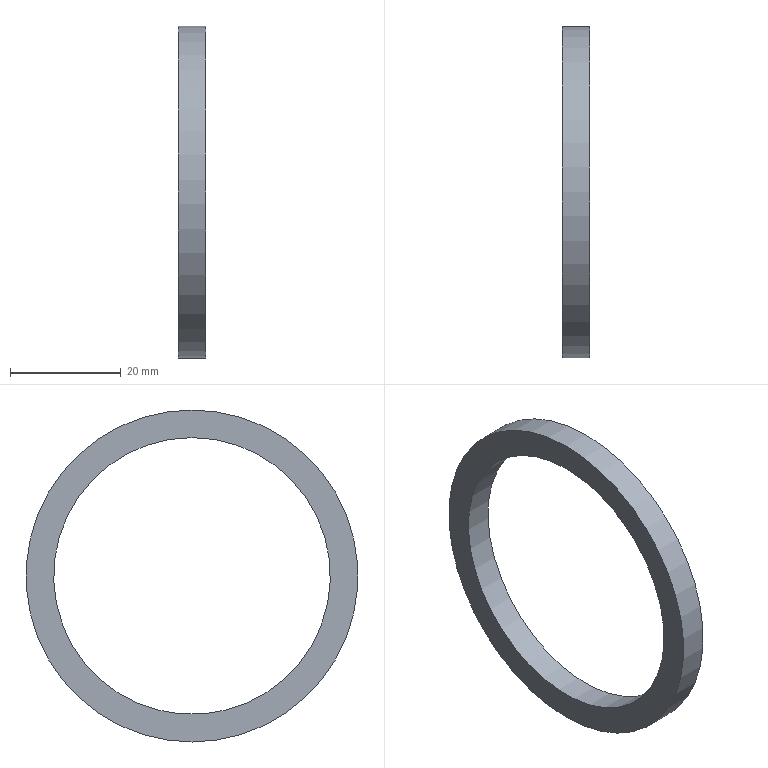Component | NX | PIN_SHAFT_WASHER | 1 solid | 4 faces | box 5 x 60 x 60 mm | volume 4320 mm3 | cylinder 2 | plane 2 | commonest cylinder face diameters 60 x1 50 x1
STEP:
#1=CARTESIAN_POINT('',(0.,0.,0.));
#2=DIRECTION('',(0.,0.,1.));
#3=DIRECTION('',(1.,0.,0.));
#4=AXIS2_PLACEMENT_3D('',#1,#2,#3);
#5=CARTESIAN_POINT('',(74.458,-1168.882,694.997));
#6=VERTEX_POINT('',#5);
#7=CARTESIAN_POINT('',(74.458,-1168.882,664.997));
#8=DIRECTION('',(1.,0.,0.));
#9=DIRECTION('',(0.,0.,1.));
#10=AXIS2_PLACEMENT_3D('',#7,#8,#9);
#11=CIRCLE('',#10,30.);
#12=CARTESIAN_POINT('',(74.458,-1168.882,664.997));
#13=DIRECTION('',(1.,0.,0.));
#14=DIRECTION('',(0.,0.,-1.));
#15=AXIS2_PLACEMENT_3D('',#12,#13,#14);
#16=CYLINDRICAL_SURFACE('',#15,30.);
#17=CARTESIAN_POINT('',(3.142,0.));
#18=DIRECTION('',(1.,0.));
#19=VECTOR('',#18,1.);
#20=LINE('',#17,#19);
#21=(GEOMETRIC_REPRESENTATION_CONTEXT(2)PARAMETRIC_REPRESENTATION_CONTEXT()REPRESENTATION_CONTEXT('',''));
#22=DEFINITIONAL_REPRESENTATION('',(#20),#21);
#23=PCURVE('',#16,#22);
#24=CARTESIAN_POINT('',(74.458,-1168.882,664.997));
#25=DIRECTION('',(1.,0.,0.));
#26=DIRECTION('',(0.,0.,-1.));
#27=AXIS2_PLACEMENT_3D('',#24,#25,#26);
#28=PLANE('',#27);
#29=CARTESIAN_POINT('',(0.,0.));
#30=DIRECTION('',(-1.,0.));
#31=AXIS2_PLACEMENT_2D('',#29,#30);
#32=CIRCLE('',#31,30.);
#33=(GEOMETRIC_REPRESENTATION_CONTEXT(2)PARAMETRIC_REPRESENTATION_CONTEXT()REPRESENTATION_CONTEXT('',''));
#34=DEFINITIONAL_REPRESENTATION('',(#32),#33);
#35=PCURVE('',#28,#34);
#36=SURFACE_CURVE('',#11,(#23,#35),.PCURVE_S1.);
#37=EDGE_CURVE('',#6,#6,#36,.T.);
#38=ORIENTED_EDGE('',*,*,#37,.T.);
#39=CARTESIAN_POINT('',(79.458,-1168.882,694.997));
#40=VERTEX_POINT('',#39);
#41=CARTESIAN_POINT('',(74.458,-1168.882,694.997));
#42=CARTESIAN_POINT('',(79.458,-1168.882,694.997));
#43=B_SPLINE_CURVE_WITH_KNOTS('',1,(#41,#42),.UNSPECIFIED.,.F.,.F.,(2,2),(0.,5.),.PIECEWISE_BEZIER_KNOTS.);
#44=CARTESIAN_POINT('',(9.425,0.));
#45=DIRECTION('',(0.,1.));
#46=VECTOR('',#45,1.);
#47=LINE('',#44,#46);
#48=(GEOMETRIC_REPRESENTATION_CONTEXT(2)PARAMETRIC_REPRESENTATION_CONTEXT()REPRESENTATION_CONTEXT('',''));
#49=DEFINITIONAL_REPRESENTATION('',(#47),#48);
#50=PCURVE('',#16,#49);
#51=CARTESIAN_POINT('',(3.142,0.));
#52=DIRECTION('',(0.,1.));
#53=VECTOR('',#52,1.);
#54=LINE('',#51,#53);
#55=(GEOMETRIC_REPRESENTATION_CONTEXT(2)PARAMETRIC_REPRESENTATION_CONTEXT()REPRESENTATION_CONTEXT('',''));
#56=DEFINITIONAL_REPRESENTATION('',(#54),#55);
#57=PCURVE('',#16,#56);
#58=SEAM_CURVE('',#43,(#50,#57),.PCURVE_S1.);
#59=EDGE_CURVE('',#6,#40,#58,.T.);
#60=ORIENTED_EDGE('',*,*,#59,.T.);
#61=CARTESIAN_POINT('',(79.458,-1168.882,664.997));
#62=DIRECTION('',(1.,0.,0.));
#63=DIRECTION('',(0.,0.,1.));
#64=AXIS2_PLACEMENT_3D('',#61,#62,#63);
#65=CIRCLE('',#64,30.);
#66=CARTESIAN_POINT('',(3.142,5.));
#67=DIRECTION('',(1.,0.));
#68=VECTOR('',#67,1.);
#69=LINE('',#66,#68);
#70=(GEOMETRIC_REPRESENTATION_CONTEXT(2)PARAMETRIC_REPRESENTATION_CONTEXT()REPRESENTATION_CONTEXT('',''));
#71=DEFINITIONAL_REPRESENTATION('',(#69),#70);
#72=PCURVE('',#16,#71);
#73=CARTESIAN_POINT('',(79.458,-1168.882,664.997));
#74=DIRECTION('',(1.,0.,0.));
#75=DIRECTION('',(0.,0.,-1.));
#76=AXIS2_PLACEMENT_3D('',#73,#74,#75);
#77=PLANE('',#76);
#78=CARTESIAN_POINT('',(0.,0.));
#79=DIRECTION('',(-1.,0.));
#80=AXIS2_PLACEMENT_2D('',#78,#79);
#81=CIRCLE('',#80,30.);
#82=(GEOMETRIC_REPRESENTATION_CONTEXT(2)PARAMETRIC_REPRESENTATION_CONTEXT()REPRESENTATION_CONTEXT('',''));
#83=DEFINITIONAL_REPRESENTATION('',(#81),#82);
#84=PCURVE('',#77,#83);
#85=SURFACE_CURVE('',#65,(#72,#84),.PCURVE_S1.);
#86=EDGE_CURVE('',#40,#40,#85,.T.);
#87=ORIENTED_EDGE('',*,*,#86,.F.);
#88=ORIENTED_EDGE('',*,*,#59,.F.);
#89=EDGE_LOOP('',(#38,#60,#87,#88));
#90=FACE_BOUND('',#89,.T.);
#91=ADVANCED_FACE('',(#90),#16,.T.);
#92=CARTESIAN_POINT('',(74.458,-1168.882,689.997));
#93=VERTEX_POINT('',#92);
#94=CARTESIAN_POINT('',(74.458,-1168.882,664.997));
#95=DIRECTION('',(1.,0.,0.));
#96=DIRECTION('',(0.,0.,1.));
#97=AXIS2_PLACEMENT_3D('',#94,#95,#96);
#98=CIRCLE('',#97,25.);
#99=CARTESIAN_POINT('',(74.458,-1168.882,664.997));
#100=DIRECTION('',(1.,0.,0.));
#101=DIRECTION('',(0.,0.,-1.));
#102=AXIS2_PLACEMENT_3D('',#99,#100,#101);
#103=CYLINDRICAL_SURFACE('',#102,25.);
#104=CARTESIAN_POINT('',(3.142,0.));
#105=DIRECTION('',(1.,0.));
#106=VECTOR('',#105,1.);
#107=LINE('',#104,#106);
#108=(GEOMETRIC_REPRESENTATION_CONTEXT(2)PARAMETRIC_REPRESENTATION_CONTEXT()REPRESENTATION_CONTEXT('',''));
#109=DEFINITIONAL_REPRESENTATION('',(#107),#108);
#110=PCURVE('',#103,#109);
#111=CARTESIAN_POINT('',(0.,0.));
#112=DIRECTION('',(-1.,0.));
#113=AXIS2_PLACEMENT_2D('',#111,#112);
#114=CIRCLE('',#113,25.);
#115=(GEOMETRIC_REPRESENTATION_CONTEXT(2)PARAMETRIC_REPRESENTATION_CONTEXT()REPRESENTATION_CONTEXT('',''));
#116=DEFINITIONAL_REPRESENTATION('',(#114),#115);
#117=PCURVE('',#28,#116);
#118=SURFACE_CURVE('',#98,(#110,#117),.PCURVE_S1.);
#119=EDGE_CURVE('',#93,#93,#118,.T.);
#120=ORIENTED_EDGE('',*,*,#119,.T.);
#121=CARTESIAN_POINT('',(79.458,-1168.882,689.997));
#122=VERTEX_POINT('',#121);
#123=CARTESIAN_POINT('',(74.458,-1168.882,689.997));
#124=CARTESIAN_POINT('',(79.458,-1168.882,689.997));
#125=B_SPLINE_CURVE_WITH_KNOTS('',1,(#123,#124),.UNSPECIFIED.,.F.,.F.,(2,2),(0.,5.),.PIECEWISE_BEZIER_KNOTS.);
#126=CARTESIAN_POINT('',(9.425,0.));
#127=DIRECTION('',(0.,1.));
#128=VECTOR('',#127,1.);
#129=LINE('',#126,#128);
#130=(GEOMETRIC_REPRESENTATION_CONTEXT(2)PARAMETRIC_REPRESENTATION_CONTEXT()REPRESENTATION_CONTEXT('',''));
#131=DEFINITIONAL_REPRESENTATION('',(#129),#130);
#132=PCURVE('',#103,#131);
#133=CARTESIAN_POINT('',(3.142,0.));
#134=DIRECTION('',(0.,1.));
#135=VECTOR('',#134,1.);
#136=LINE('',#133,#135);
#137=(GEOMETRIC_REPRESENTATION_CONTEXT(2)PARAMETRIC_REPRESENTATION_CONTEXT()REPRESENTATION_CONTEXT('',''));
#138=DEFINITIONAL_REPRESENTATION('',(#136),#137);
#139=PCURVE('',#103,#138);
#140=SEAM_CURVE('',#125,(#132,#139),.PCURVE_S1.);
#141=EDGE_CURVE('',#93,#122,#140,.T.);
#142=ORIENTED_EDGE('',*,*,#141,.T.);
#143=CARTESIAN_POINT('',(79.458,-1168.882,664.997));
#144=DIRECTION('',(1.,0.,0.));
#145=DIRECTION('',(0.,0.,1.));
#146=AXIS2_PLACEMENT_3D('',#143,#144,#145);
#147=CIRCLE('',#146,25.);
#148=CARTESIAN_POINT('',(3.142,5.));
#149=DIRECTION('',(1.,0.));
#150=VECTOR('',#149,1.);
#151=LINE('',#148,#150);
#152=(GEOMETRIC_REPRESENTATION_CONTEXT(2)PARAMETRIC_REPRESENTATION_CONTEXT()REPRESENTATION_CONTEXT('',''));
#153=DEFINITIONAL_REPRESENTATION('',(#151),#152);
#154=PCURVE('',#103,#153);
#155=CARTESIAN_POINT('',(0.,0.));
#156=DIRECTION('',(-1.,0.));
#157=AXIS2_PLACEMENT_2D('',#155,#156);
#158=CIRCLE('',#157,25.);
#159=(GEOMETRIC_REPRESENTATION_CONTEXT(2)PARAMETRIC_REPRESENTATION_CONTEXT()REPRESENTATION_CONTEXT('',''));
#160=DEFINITIONAL_REPRESENTATION('',(#158),#159);
#161=PCURVE('',#77,#160);
#162=SURFACE_CURVE('',#147,(#154,#161),.PCURVE_S1.);
#163=EDGE_CURVE('',#122,#122,#162,.T.);
#164=ORIENTED_EDGE('',*,*,#163,.F.);
#165=ORIENTED_EDGE('',*,*,#141,.F.);
#166=EDGE_LOOP('',(#120,#142,#164,#165));
#167=FACE_BOUND('',#166,.F.);
#168=ADVANCED_FACE('',(#167),#103,.F.);
#169=ORIENTED_EDGE('',*,*,#37,.F.);
#170=EDGE_LOOP('',(#169));
#171=FACE_BOUND('',#170,.T.);
#172=ORIENTED_EDGE('',*,*,#119,.T.);
#173=EDGE_LOOP('',(#172));
#174=FACE_BOUND('',#173,.T.);
#175=ADVANCED_FACE('',(#171,#174),#28,.F.);
#176=ORIENTED_EDGE('',*,*,#86,.T.);
#177=EDGE_LOOP('',(#176));
#178=FACE_BOUND('',#177,.T.);
#179=ORIENTED_EDGE('',*,*,#163,.F.);
#180=EDGE_LOOP('',(#179));
#181=FACE_BOUND('',#180,.T.);
#182=ADVANCED_FACE('',(#178,#181),#77,.T.);
#183=CLOSED_SHELL('',(#91,#168,#175,#182));
#184=MANIFOLD_SOLID_BREP('',#183);
#185=(LENGTH_UNIT()NAMED_UNIT(*)SI_UNIT(.MILLI.,.METRE.));
#186=UNCERTAINTY_MEASURE_WITH_UNIT(LENGTH_MEASURE(0.00001),#185,'','');
#187=(NAMED_UNIT(*)PLANE_ANGLE_UNIT()SI_UNIT($,.RADIAN.));
#188=(NAMED_UNIT(*)SI_UNIT($,.STERADIAN.)SOLID_ANGLE_UNIT());
#189=(GEOMETRIC_REPRESENTATION_CONTEXT(3)GLOBAL_UNCERTAINTY_ASSIGNED_CONTEXT((#186))GLOBAL_UNIT_ASSIGNED_CONTEXT((#185,#187,#188))REPRESENTATION_CONTEXT('',''));
#190=ADVANCED_BREP_SHAPE_REPRESENTATION('',(#4,#184),#189);